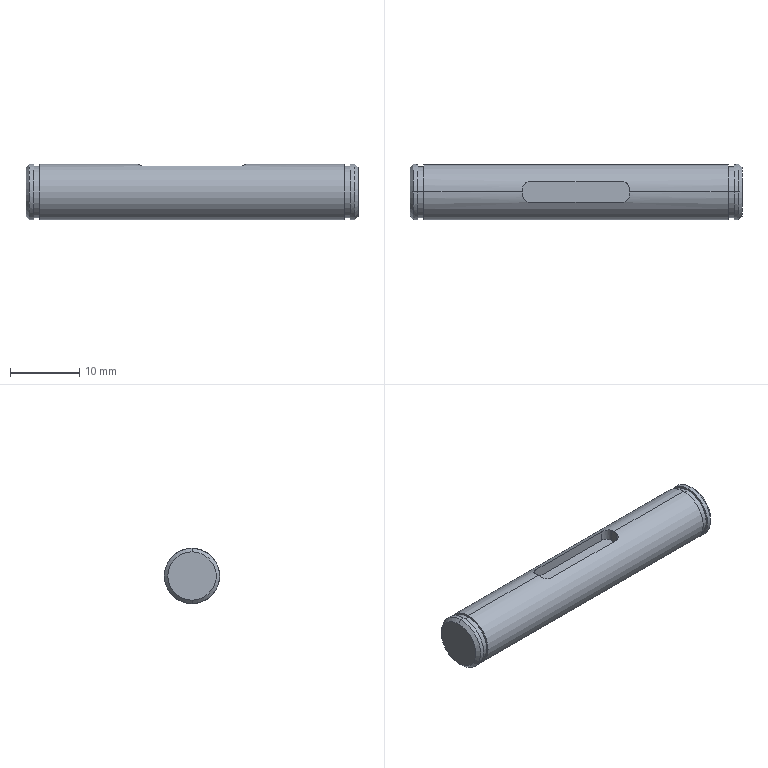CAM job | Mastercam | mm | 3 operations | part box 48 x 8 x 8
1. Contour (Ramp) | 1 - 2 平铣刀
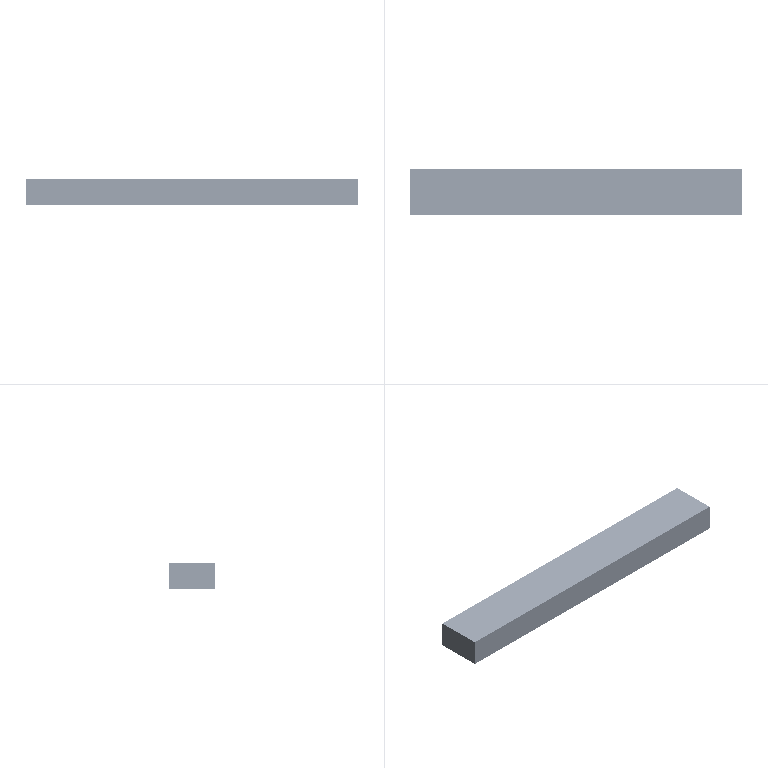2. Contour (2D) | 2 - 2 平铣刀
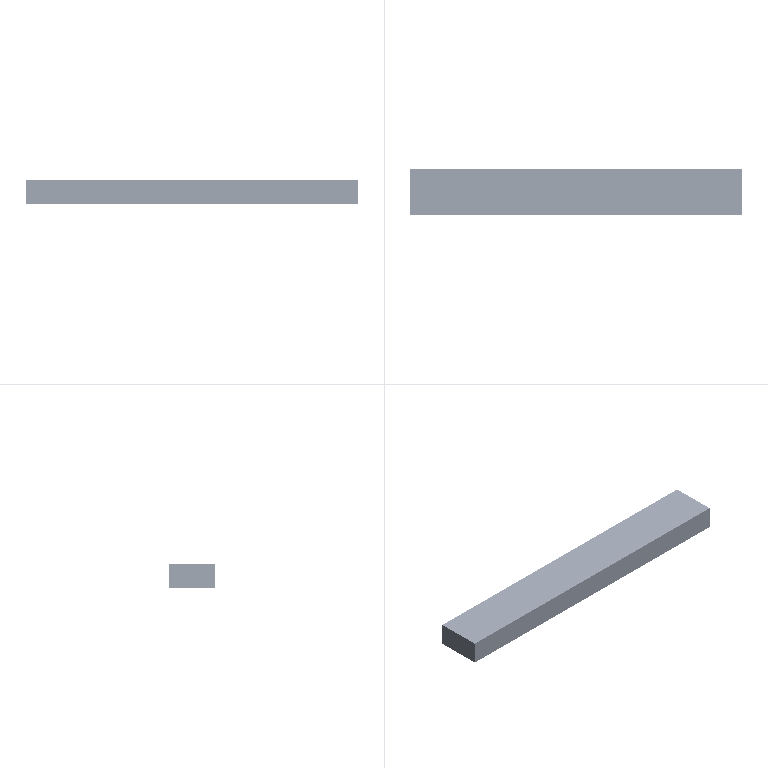3. Contour (3D chamfer) | 3 - 4 倒角刀